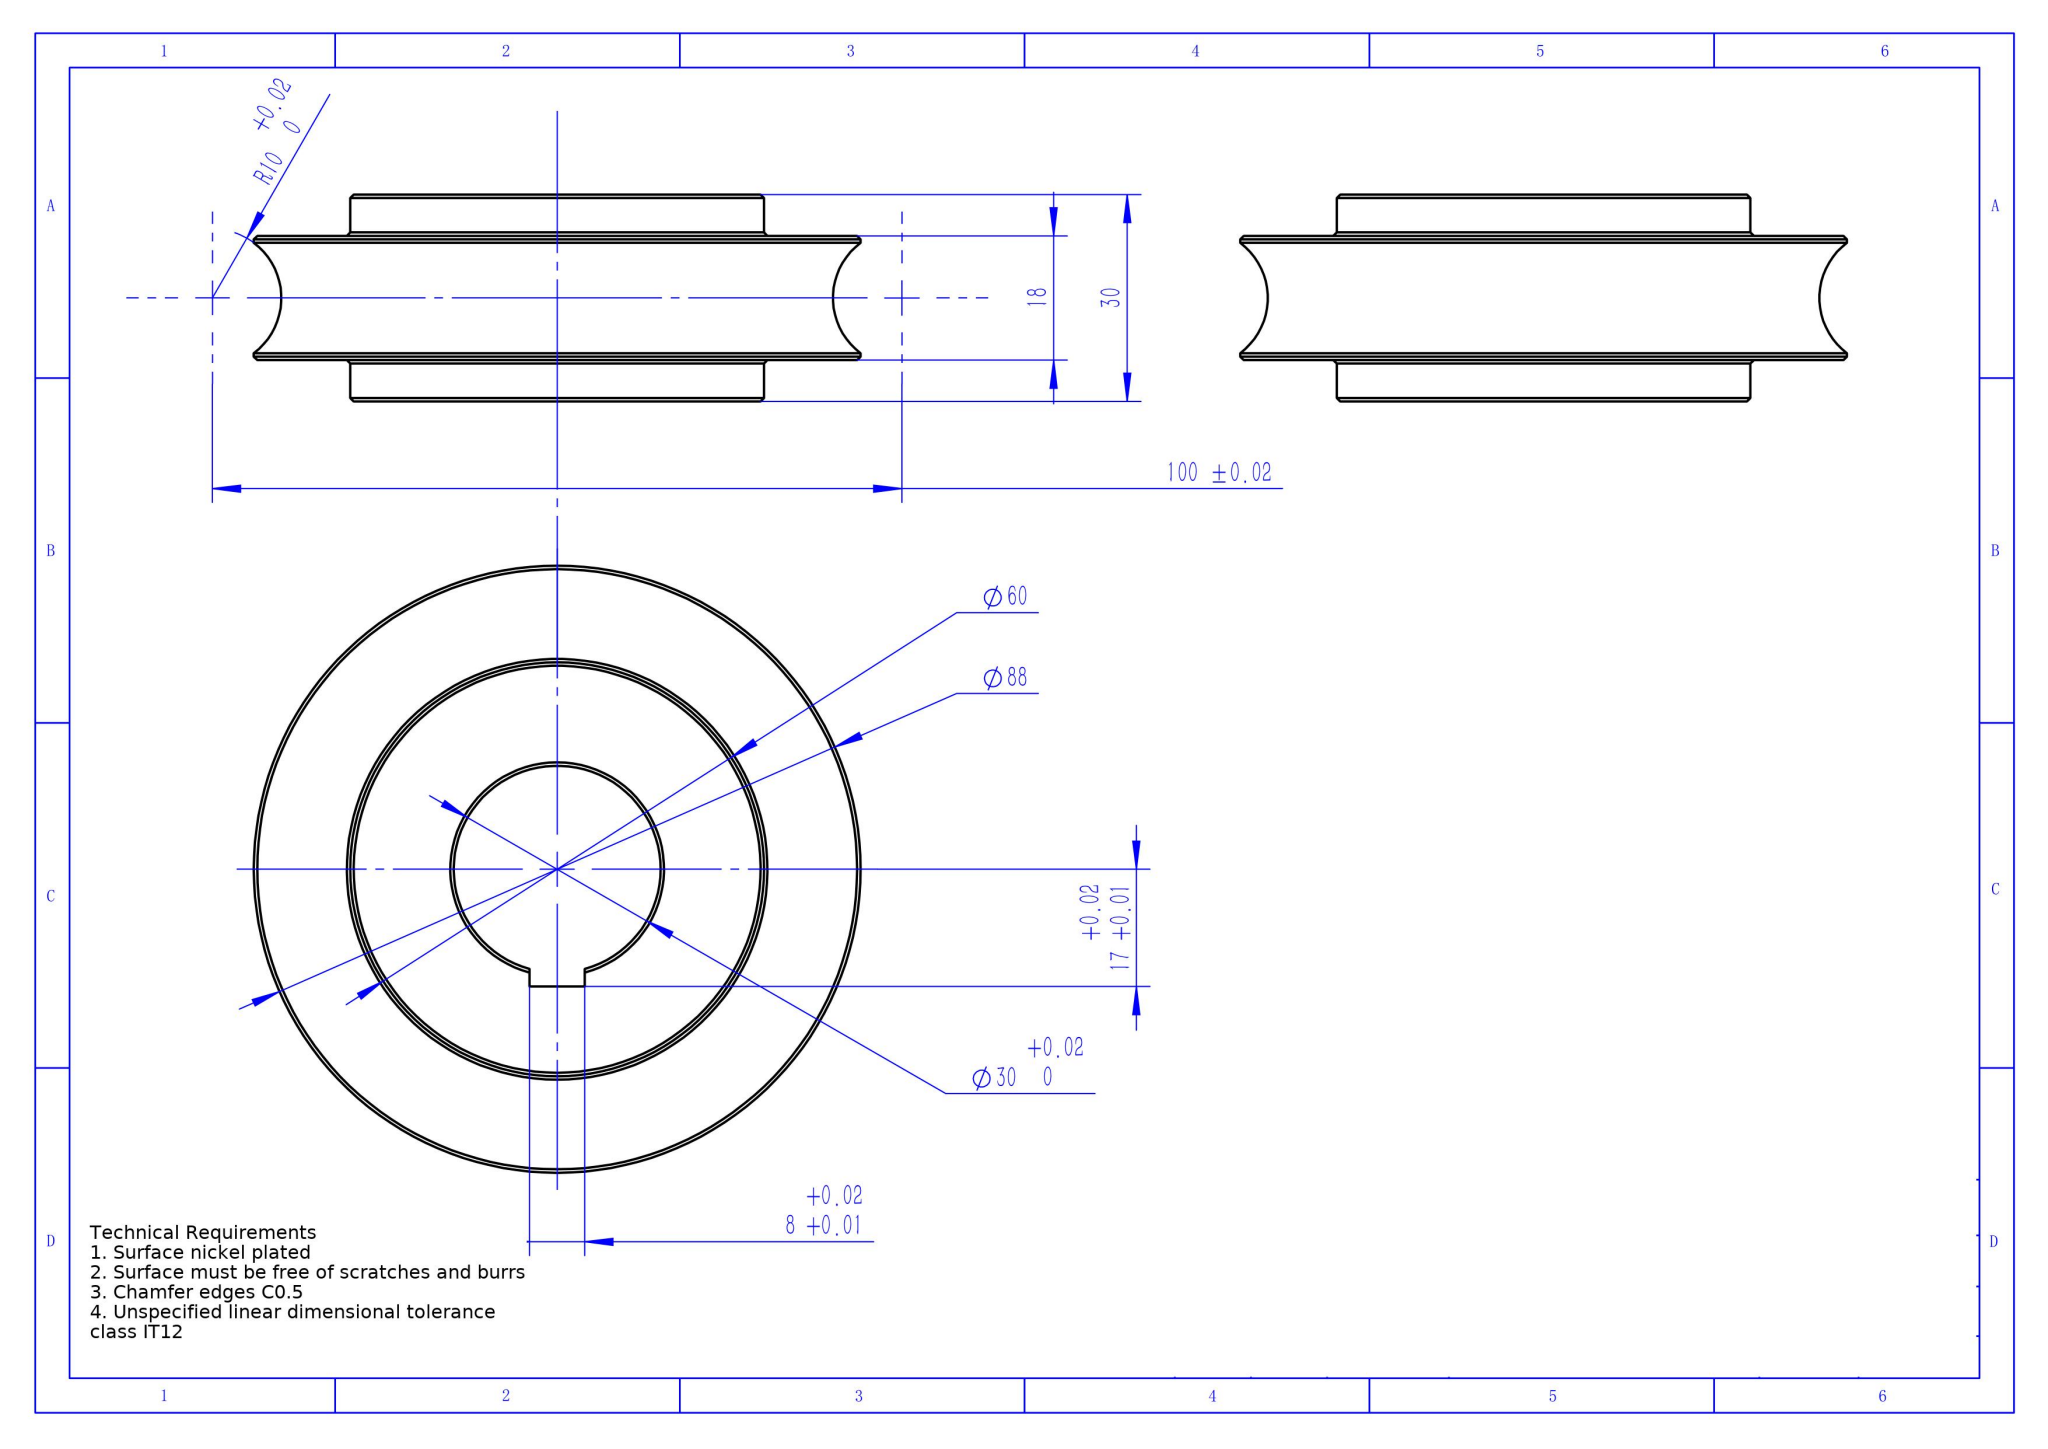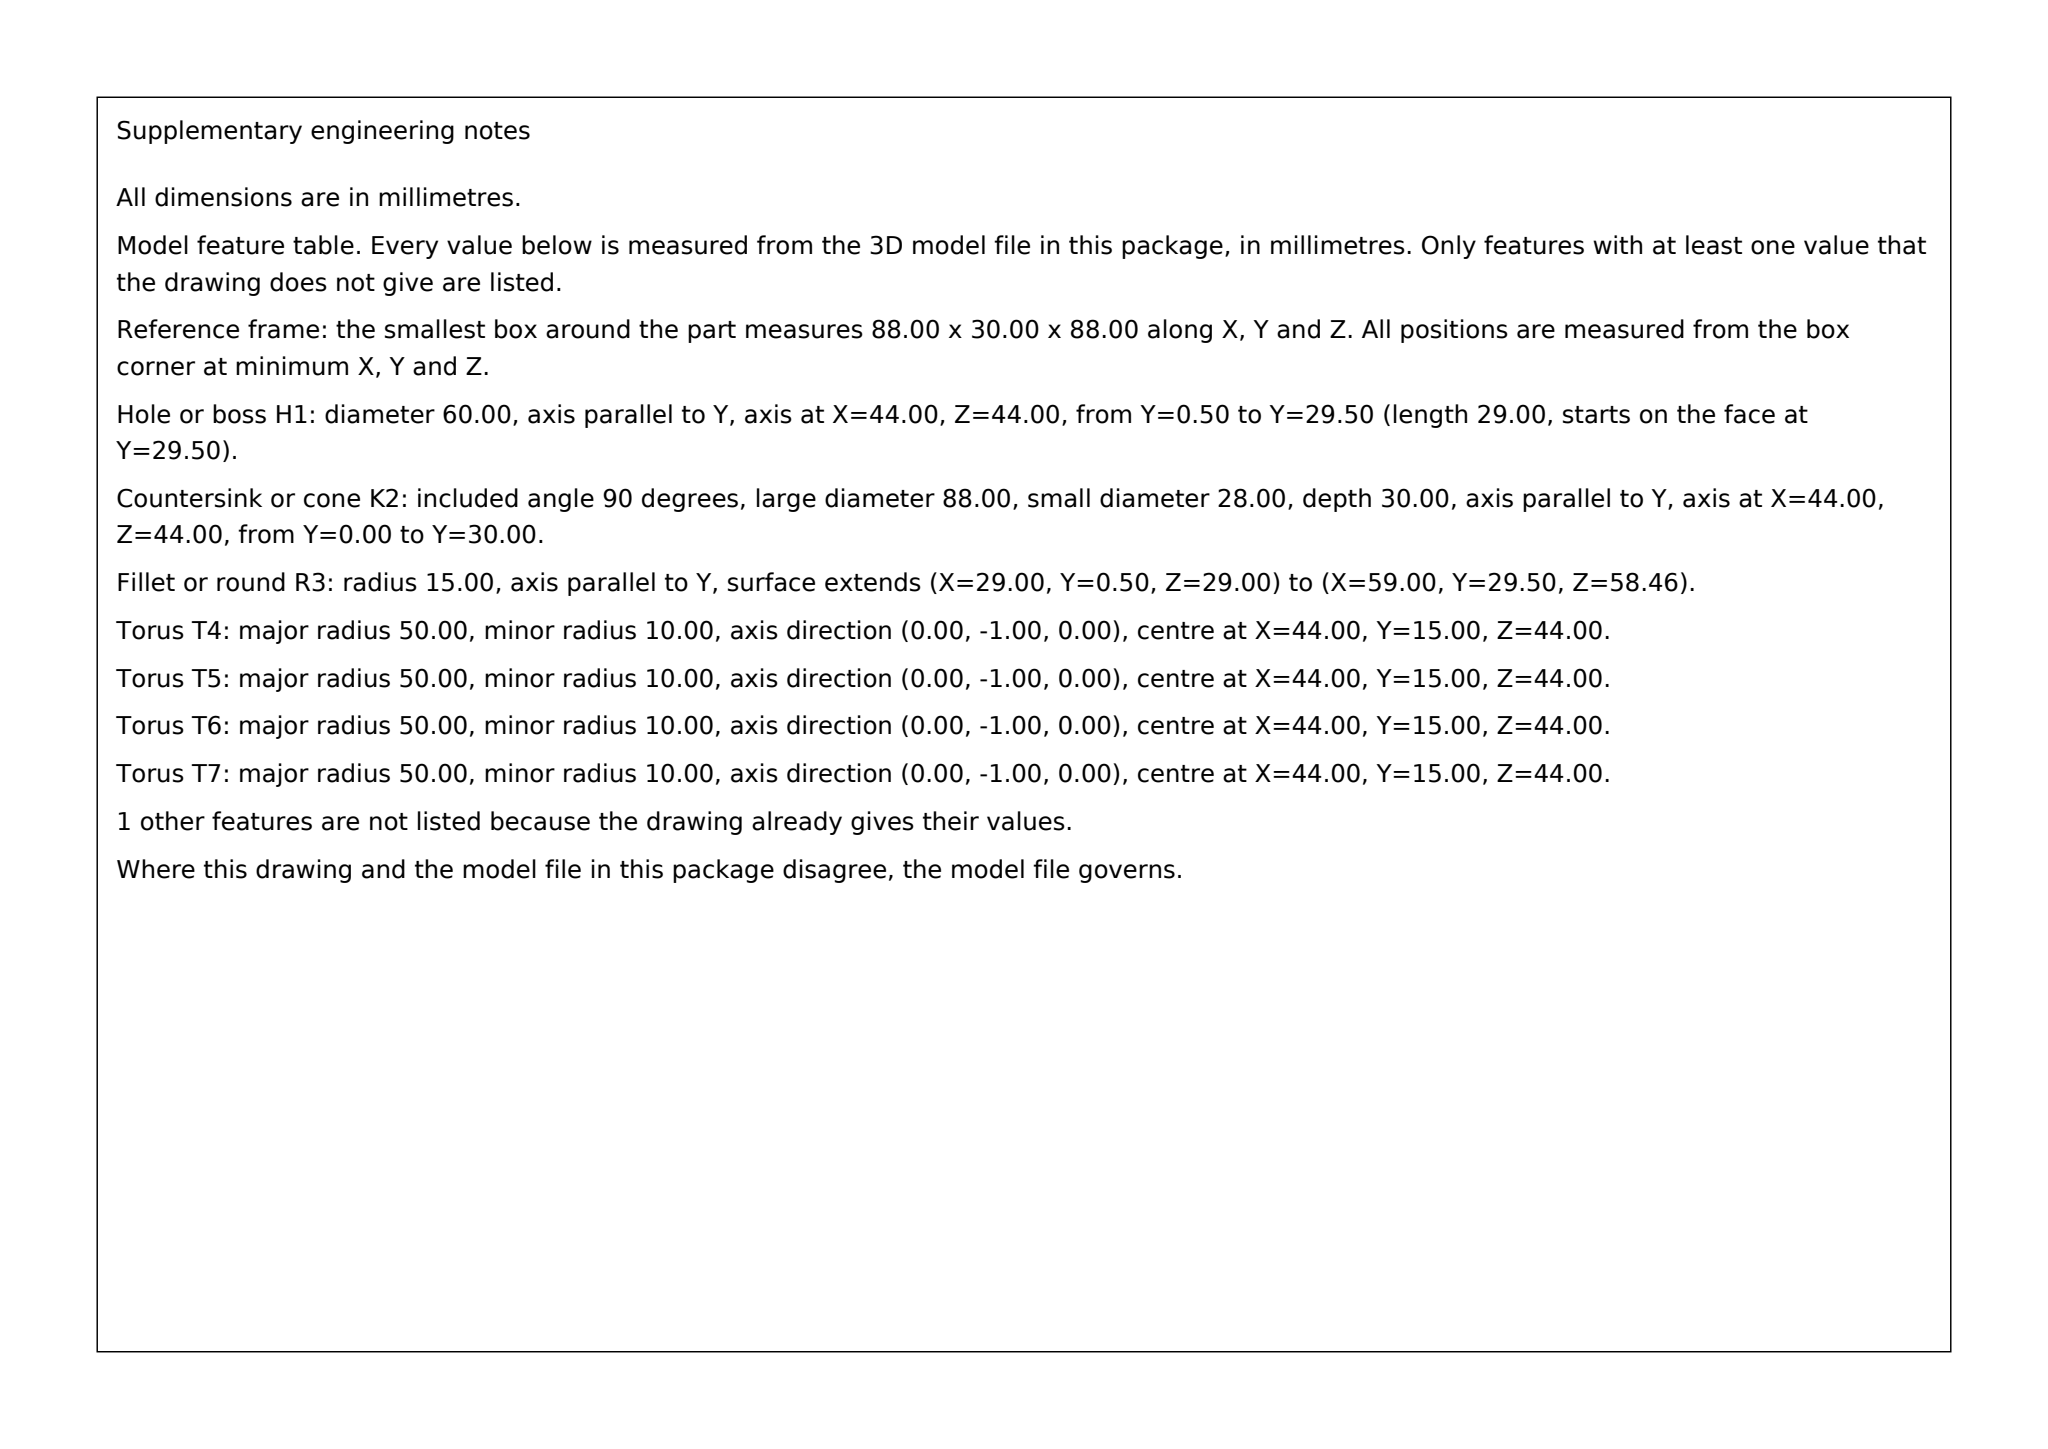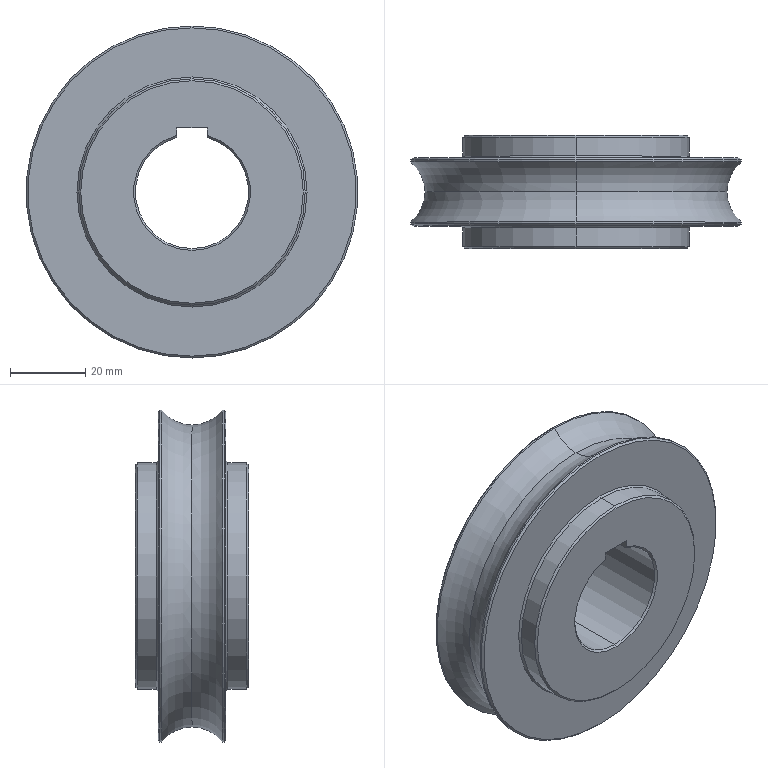Part | SolidWorks | mm | 1 solid | 36 faces | box 88 x 30 x 88 mm | volume 109681 mm3 | cone 15 | cylinder 10 | plane 7 | torus 4 | commonest cylinder face diameters 60 x4 88 x4 30 x2
build123d program:
from build123d import *

# Parameters (mm, degrees)
CHAMFER1_SIZE = 0.5
KEYWAY_DEPTH  = 88.699


with BuildPart() as part:
    # Sketch1 → Revolve1 (revolve)
    with BuildSketch(Plane.XY, mode=Mode.PRIVATE) as revolve1_sk:
        with BuildLine():
            Line((15, -15), (30, -15))
            Line((30, -15), (30, -9))
            Line((30, -9), (44, -9))
            Line((44, -9), (44, -8))
            ThreePointArc((44, -8), (40, 0), (44, 8))
            Line((44, 8), (44, 9))
            Line((44, 9), (30, 9))
            Line((30, 9), (30, 15))
            Line((30, 15), (15, 15))
            Line((15, 15), (15, -15))
        make_face()
    revolve(revolve1_sk.sketch.rotate(Axis((0, 0, 0), (0, 1, 0)), 90), axis=Axis((0, 0, 0), (0, 1, 0)))

    # Chamfer1
    chamfer1_edges = [part.edges().sort_by_distance(p)[0] for p in [
        (0, -9, 44),
        (0, -9, 30),
        (0, -15, 30),
        (0, -15, 15),
        (0, 15, 15),
        (0, 15, 30),
        (0, 9, 30),
        (0, 9, 44),
    ]]
    chamfer(chamfer1_edges, length=CHAMFER1_SIZE)

    # KeySketch → Keyway (cut, through all)
    with BuildSketch(Plane(origin=(17.778, 15, -10.539), x_dir=(-1, 0, 0), z_dir=(0, 1, 0))):
        with BuildLine():
            Line((13.778, 24.996), (13.778, 27.539))
            Line((13.778, 27.539), (21.778, 27.539))
            Line((21.778, 27.539), (21.778, 24.996))
            ThreePointArc((21.778, 24.996), (17.778, -4.461), (13.778, 24.996))
        make_face()
    extrude(amount=-KEYWAY_DEPTH, mode=Mode.SUBTRACT)


solid = part.part